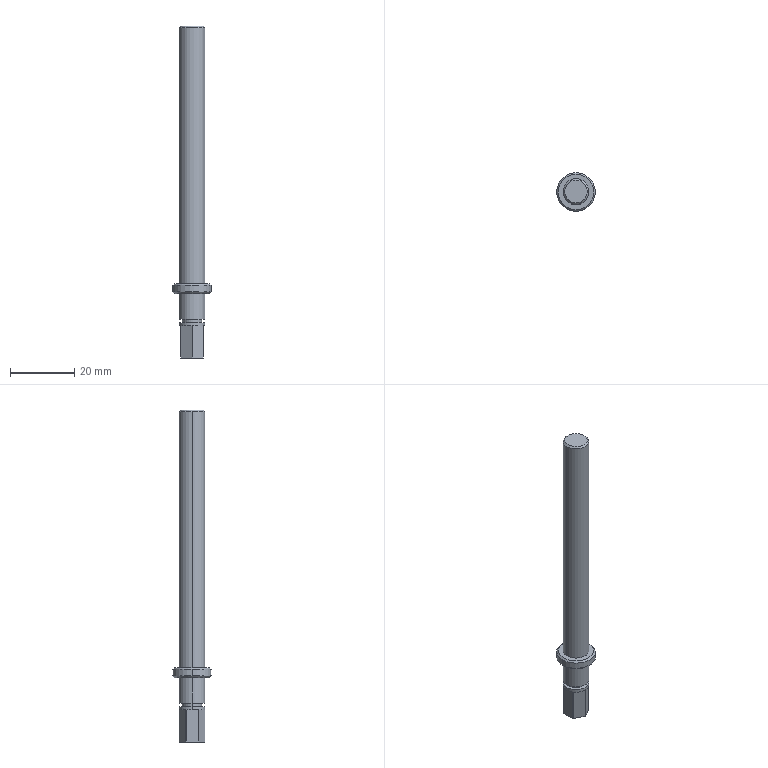CAM job | Mastercam | mm | 1 operations | part box 12 x 12 x 103
1. Contour (Ramp) | 15 - 12 平铣刀